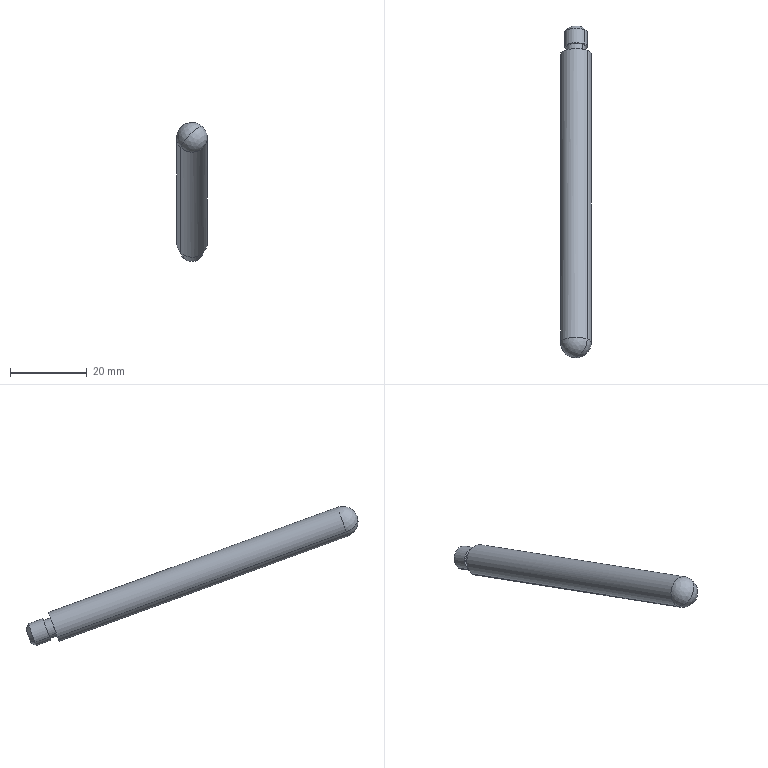Component | SolidWorks | Bipod-1 | 1 solid | 13 faces | box 8 x 86.44 x 36.23 mm | volume 4328 mm3 | cylinder 6 | plane 3 | cone 2 | sphere 2 | commonest cylinder face diameters 8 x2 5 x2 6 x2
build123d program:
from build123d import *

# Parameters (mm, degrees)
FILLET1_R     = 4
CHAMFER1_SIZE = 1


with BuildPart() as part:
    # Sketch1 → Revolve1 (revolve)
    with BuildSketch(Plane.XY, mode=Mode.PRIVATE) as revolve1_sk:
        Polygon((0, 0), (0, 3), (5, 3), (5, 2.5), (7, 2.5), (7, 4), (91, 4), (91, 0), align=None)
    revolve(revolve1_sk.sketch.rotate(Axis((0, 0, 0), (1, 0, 0)), 90), axis=Axis((0, 0, 0), (1, 0, 0)))

    # Fillet1
    fillet1_edges = [part.edges().sort_by_distance(p)[0] for p in [
        (91, 0, -4),
    ]]
    fillet(fillet1_edges, radius=FILLET1_R)

    # Chamfer1
    chamfer1_edges = [part.edges().sort_by_distance(p)[0] for p in [
        (0, 0, -3),
    ]]
    chamfer(chamfer1_edges, length=CHAMFER1_SIZE)


solid = part.part

# Placed as in the assembly
solid = solid.moved(Location((-140.818, 19.624, 1018.001), (160, 0.8472, 90)))
STEP:
#1=CARTESIAN_POINT('',(-5.601,0.7541,40.028));
#2=VERTEX_POINT('',#1);
#3=CARTESIAN_POINT('',(-5.487,0.7911,40.13));
#4=VERTEX_POINT('',#3);
#5=CARTESIAN_POINT('',(-5.544,0.7726,40.079));
#6=DIRECTION('',(-0.,0.9397,-0.342));
#7=DIRECTION('',(0.7279,0.2345,0.6444));
#8=AXIS2_PLACEMENT_3D('',#5,#6,#7);
#9=CIRCLE('',#8,0.07874);
#10=EDGE_CURVE('',#2,#4,#9,.T.);
#11=ORIENTED_EDGE('',*,*,#10,.F.);
#12=CARTESIAN_POINT('',(-5.63,0.7079,40.016));
#13=VERTEX_POINT('',#12);
#14=CARTESIAN_POINT('',(-5.601,0.7541,40.028));
#15=DIRECTION('',(-0.5147,-0.8303,-0.2138));
#16=VECTOR('',#15,39.37);
#17=LINE('',#14,#16);
#18=EDGE_CURVE('',#2,#13,#17,.T.);
#19=ORIENTED_EDGE('',*,*,#18,.T.);
#20=CARTESIAN_POINT('',(-5.458,0.7633,40.168));
#21=VERTEX_POINT('',#20);
#22=CARTESIAN_POINT('',(-5.544,0.7356,40.092));
#23=DIRECTION('',(0.,-0.9397,0.342));
#24=DIRECTION('',(0.7279,0.2345,0.6444));
#25=AXIS2_PLACEMENT_3D('',#22,#23,#24);
#26=CIRCLE('',#25,0.1181);
#27=EDGE_CURVE('',#21,#13,#26,.T.);
#28=ORIENTED_EDGE('',*,*,#27,.F.);
#29=CARTESIAN_POINT('',(-5.487,0.7911,40.13));
#30=DIRECTION('',(0.5147,-0.4986,0.6975));
#31=VECTOR('',#30,39.37);
#32=LINE('',#29,#31);
#33=EDGE_CURVE('',#4,#21,#32,.T.);
#34=ORIENTED_EDGE('',*,*,#33,.F.);
#35=EDGE_LOOP('',(#11,#19,#28,#34));
#36=FACE_OUTER_BOUND('',#35,.T.);
#37=CARTESIAN_POINT('',(-5.544,0.7726,40.079));
#38=DIRECTION('',(0.,-0.9397,0.342));
#39=DIRECTION('',(0.7279,0.2345,0.6444));
#40=AXIS2_PLACEMENT_3D('',#37,#38,#39);
#41=CONICAL_SURFACE('',#40,0.07874,0.7854);
#42=ADVANCED_FACE('',(#36),#41,.T.);
#43=CARTESIAN_POINT('',(-5.544,-2.594,41.304));
#44=VERTEX_POINT('',#43);
#45=CARTESIAN_POINT('',(-5.659,-2.483,41.149));
#46=VERTEX_POINT('',#45);
#47=CARTESIAN_POINT('',(-5.544,-2.446,41.25));
#48=DIRECTION('',(0.6857,-0.2489,-0.684));
#49=DIRECTION('',(-0.7062,0.,-0.708));
#50=AXIS2_PLACEMENT_3D('',#47,#48,#49);
#51=CIRCLE('',#50,0.1575);
#52=EDGE_CURVE('',#44,#46,#51,.T.);
#53=ORIENTED_EDGE('',*,*,#52,.F.);
#54=CARTESIAN_POINT('',(-5.429,-2.409,41.352));
#55=VERTEX_POINT('',#54);
#56=CARTESIAN_POINT('',(-5.544,-2.446,41.25));
#57=DIRECTION('',(-0.6857,0.2489,0.684));
#58=DIRECTION('',(0.7062,0.,0.708));
#59=AXIS2_PLACEMENT_3D('',#56,#57,#58);
#60=CIRCLE('',#59,0.1575);
#61=EDGE_CURVE('',#44,#55,#60,.T.);
#62=ORIENTED_EDGE('',*,*,#61,.T.);
#63=CARTESIAN_POINT('',(-5.544,-2.446,41.25));
#64=DIRECTION('',(-0.,0.9397,-0.342));
#65=DIRECTION('',(-0.7279,-0.2345,-0.6444));
#66=AXIS2_PLACEMENT_3D('',#63,#64,#65);
#67=CIRCLE('',#66,0.1575);
#68=EDGE_CURVE('',#46,#55,#67,.T.);
#69=ORIENTED_EDGE('',*,*,#68,.F.);
#70=EDGE_LOOP('',(#53,#62,#69));
#71=FACE_OUTER_BOUND('',#70,.T.);
#72=CARTESIAN_POINT('',(-5.544,-2.446,41.25));
#73=DIRECTION('',(-0.6857,0.2489,0.684));
#74=DIRECTION('',(-0.7279,-0.2345,-0.6444));
#75=AXIS2_PLACEMENT_3D('',#72,#73,#74);
#76=SPHERICAL_SURFACE('',#75,0.1575);
#77=ADVANCED_FACE('',(#71),#76,.T.);
#78=ORIENTED_EDGE('',*,*,#68,.T.);
#79=CARTESIAN_POINT('',(-5.429,0.5506,40.275));
#80=VERTEX_POINT('',#79);
#81=CARTESIAN_POINT('',(-5.429,0.8095,40.18));
#82=DIRECTION('',(-0.,0.9397,-0.342));
#83=VECTOR('',#82,39.37);
#84=LINE('',#81,#83);
#85=EDGE_CURVE('',#55,#80,#84,.T.);
#86=ORIENTED_EDGE('',*,*,#85,.T.);
#87=CARTESIAN_POINT('',(-5.659,0.4767,40.072));
#88=VERTEX_POINT('',#87);
#89=CARTESIAN_POINT('',(-5.544,0.5136,40.173));
#90=DIRECTION('',(-0.,0.9397,-0.342));
#91=DIRECTION('',(-0.7279,-0.2345,-0.6444));
#92=AXIS2_PLACEMENT_3D('',#89,#90,#91);
#93=CIRCLE('',#92,0.1575);
#94=EDGE_CURVE('',#88,#80,#93,.T.);
#95=ORIENTED_EDGE('',*,*,#94,.F.);
#96=CARTESIAN_POINT('',(-5.659,0.7357,39.977));
#97=DIRECTION('',(-0.,0.9397,-0.342));
#98=VECTOR('',#97,39.37);
#99=LINE('',#96,#98);
#100=EDGE_CURVE('',#46,#88,#99,.T.);
#101=ORIENTED_EDGE('',*,*,#100,.F.);
#102=EDGE_LOOP('',(#78,#86,#95,#101));
#103=FACE_OUTER_BOUND('',#102,.T.);
#104=CARTESIAN_POINT('',(-5.544,0.7726,40.079));
#105=DIRECTION('',(-0.,0.9397,-0.342));
#106=DIRECTION('',(-0.7279,-0.2345,-0.6444));
#107=AXIS2_PLACEMENT_3D('',#104,#105,#106);
#108=CYLINDRICAL_SURFACE('',#107,0.1575);
#109=ADVANCED_FACE('',(#103),#108,.T.);
#110=CARTESIAN_POINT('',(-5.616,0.4905,40.11));
#111=VERTEX_POINT('',#110);
#112=CARTESIAN_POINT('',(-5.472,0.5367,40.236));
#113=VERTEX_POINT('',#112);
#114=CARTESIAN_POINT('',(-5.544,0.5136,40.173));
#115=DIRECTION('',(-0.,0.9397,-0.342));
#116=DIRECTION('',(-0.7279,-0.2345,-0.6444));
#117=AXIS2_PLACEMENT_3D('',#114,#115,#116);
#118=CIRCLE('',#117,0.09843);
#119=EDGE_CURVE('',#111,#113,#118,.T.);
#120=ORIENTED_EDGE('',*,*,#119,.T.);
#121=CARTESIAN_POINT('',(-5.472,0.6107,40.21));
#122=VERTEX_POINT('',#121);
#123=CARTESIAN_POINT('',(-5.472,0.7957,40.142));
#124=DIRECTION('',(-0.,0.9397,-0.342));
#125=VECTOR('',#124,39.37);
#126=LINE('',#123,#125);
#127=EDGE_CURVE('',#113,#122,#126,.T.);
#128=ORIENTED_EDGE('',*,*,#127,.T.);
#129=CARTESIAN_POINT('',(-5.616,0.5645,40.083));
#130=VERTEX_POINT('',#129);
#131=CARTESIAN_POINT('',(-5.544,0.5876,40.146));
#132=DIRECTION('',(-0.,0.9397,-0.342));
#133=DIRECTION('',(-0.7279,-0.2345,-0.6444));
#134=AXIS2_PLACEMENT_3D('',#131,#132,#133);
#135=CIRCLE('',#134,0.09843);
#136=EDGE_CURVE('',#130,#122,#135,.T.);
#137=ORIENTED_EDGE('',*,*,#136,.F.);
#138=CARTESIAN_POINT('',(-5.616,0.7495,40.015));
#139=DIRECTION('',(-0.,0.9397,-0.342));
#140=VECTOR('',#139,39.37);
#141=LINE('',#138,#140);
#142=EDGE_CURVE('',#111,#130,#141,.T.);
#143=ORIENTED_EDGE('',*,*,#142,.F.);
#144=EDGE_LOOP('',(#120,#128,#137,#143));
#145=FACE_OUTER_BOUND('',#144,.T.);
#146=CARTESIAN_POINT('',(-5.544,0.7726,40.079));
#147=DIRECTION('',(-0.,0.9397,-0.342));
#148=DIRECTION('',(-0.7279,-0.2345,-0.6444));
#149=AXIS2_PLACEMENT_3D('',#146,#147,#148);
#150=CYLINDRICAL_SURFACE('',#149,0.09843);
#151=ADVANCED_FACE('',(#145),#150,.T.);
#152=CARTESIAN_POINT('',(-5.63,0.5599,40.07));
#153=VERTEX_POINT('',#152);
#154=CARTESIAN_POINT('',(-5.458,0.6153,40.222));
#155=VERTEX_POINT('',#154);
#156=CARTESIAN_POINT('',(-5.544,0.5876,40.146));
#157=DIRECTION('',(-0.,0.9397,-0.342));
#158=DIRECTION('',(-0.7279,-0.2345,-0.6444));
#159=AXIS2_PLACEMENT_3D('',#156,#157,#158);
#160=CIRCLE('',#159,0.1181);
#161=EDGE_CURVE('',#153,#155,#160,.T.);
#162=ORIENTED_EDGE('',*,*,#161,.T.);
#163=CARTESIAN_POINT('',(-5.458,0.8003,40.155));
#164=DIRECTION('',(-0.,0.9397,-0.342));
#165=VECTOR('',#164,39.37);
#166=LINE('',#163,#165);
#167=EDGE_CURVE('',#155,#21,#166,.T.);
#168=ORIENTED_EDGE('',*,*,#167,.T.);
#169=ORIENTED_EDGE('',*,*,#27,.T.);
#170=CARTESIAN_POINT('',(-5.63,0.7449,40.003));
#171=DIRECTION('',(-0.,0.9397,-0.342));
#172=VECTOR('',#171,39.37);
#173=LINE('',#170,#172);
#174=EDGE_CURVE('',#153,#13,#173,.T.);
#175=ORIENTED_EDGE('',*,*,#174,.F.);
#176=EDGE_LOOP('',(#162,#168,#169,#175));
#177=FACE_OUTER_BOUND('',#176,.T.);
#178=CARTESIAN_POINT('',(-5.544,0.7726,40.079));
#179=DIRECTION('',(-0.,0.9397,-0.342));
#180=DIRECTION('',(-0.7279,-0.2345,-0.6444));
#181=AXIS2_PLACEMENT_3D('',#178,#179,#180);
#182=CYLINDRICAL_SURFACE('',#181,0.1181);
#183=ADVANCED_FACE('',(#177),#182,.T.);
#184=CARTESIAN_POINT('',(-5.544,0.7726,40.079));
#185=DIRECTION('',(-0.,0.9397,-0.342));
#186=DIRECTION('',(0.7279,0.2345,0.6444));
#187=AXIS2_PLACEMENT_3D('',#184,#185,#186);
#188=CIRCLE('',#187,0.07874);
#189=EDGE_CURVE('',#4,#2,#188,.T.);
#190=ORIENTED_EDGE('',*,*,#189,.T.);
#191=ORIENTED_EDGE('',*,*,#10,.T.);
#192=EDGE_LOOP('',(#190,#191));
#193=FACE_OUTER_BOUND('',#192,.T.);
#194=CARTESIAN_POINT('',(-5.544,0.7726,40.079));
#195=DIRECTION('',(-0.,-0.9397,0.342));
#196=DIRECTION('',(0.7279,0.2345,0.6444));
#197=AXIS2_PLACEMENT_3D('',#194,#195,#196);
#198=PLANE('',#197);
#199=ADVANCED_FACE('',(#193),#198,.F.);
#200=ORIENTED_EDGE('',*,*,#167,.F.);
#201=CARTESIAN_POINT('',(-5.544,0.5876,40.146));
#202=DIRECTION('',(-0.,0.9397,-0.342));
#203=DIRECTION('',(-0.7279,-0.2345,-0.6444));
#204=AXIS2_PLACEMENT_3D('',#201,#202,#203);
#205=CIRCLE('',#204,0.1181);
#206=EDGE_CURVE('',#155,#153,#205,.T.);
#207=ORIENTED_EDGE('',*,*,#206,.T.);
#208=ORIENTED_EDGE('',*,*,#174,.T.);
#209=CARTESIAN_POINT('',(-5.544,0.7356,40.092));
#210=DIRECTION('',(0.,-0.9397,0.342));
#211=DIRECTION('',(0.7279,0.2345,0.6444));
#212=AXIS2_PLACEMENT_3D('',#209,#210,#211);
#213=CIRCLE('',#212,0.1181);
#214=EDGE_CURVE('',#13,#21,#213,.T.);
#215=ORIENTED_EDGE('',*,*,#214,.T.);
#216=EDGE_LOOP('',(#200,#207,#208,#215));
#217=FACE_OUTER_BOUND('',#216,.T.);
#218=CARTESIAN_POINT('',(-5.544,0.7726,40.079));
#219=DIRECTION('',(-0.,0.9397,-0.342));
#220=DIRECTION('',(-0.7279,-0.2345,-0.6444));
#221=AXIS2_PLACEMENT_3D('',#218,#219,#220);
#222=CYLINDRICAL_SURFACE('',#221,0.1181);
#223=ADVANCED_FACE('',(#217),#222,.T.);
#224=ORIENTED_EDGE('',*,*,#161,.F.);
#225=ORIENTED_EDGE('',*,*,#206,.F.);
#226=EDGE_LOOP('',(#224,#225));
#227=FACE_OUTER_BOUND('',#226,.T.);
#228=ORIENTED_EDGE('',*,*,#136,.T.);
#229=CARTESIAN_POINT('',(-5.544,0.5876,40.146));
#230=DIRECTION('',(-0.,0.9397,-0.342));
#231=DIRECTION('',(-0.7279,-0.2345,-0.6444));
#232=AXIS2_PLACEMENT_3D('',#229,#230,#231);
#233=CIRCLE('',#232,0.09843);
#234=EDGE_CURVE('',#122,#130,#233,.T.);
#235=ORIENTED_EDGE('',*,*,#234,.T.);
#236=EDGE_LOOP('',(#228,#235));
#237=FACE_BOUND('',#236,.T.);
#238=CARTESIAN_POINT('',(-5.625,0.617,40.227));
#239=DIRECTION('',(0.,0.9397,-0.342));
#240=DIRECTION('',(-0.7279,-0.2345,-0.6444));
#241=AXIS2_PLACEMENT_3D('',#238,#239,#240);
#242=PLANE('',#241);
#243=ADVANCED_FACE('',(#227,#237),#242,.F.);
#244=ORIENTED_EDGE('',*,*,#127,.F.);
#245=CARTESIAN_POINT('',(-5.544,0.5136,40.173));
#246=DIRECTION('',(-0.,0.9397,-0.342));
#247=DIRECTION('',(-0.7279,-0.2345,-0.6444));
#248=AXIS2_PLACEMENT_3D('',#245,#246,#247);
#249=CIRCLE('',#248,0.09843);
#250=EDGE_CURVE('',#113,#111,#249,.T.);
#251=ORIENTED_EDGE('',*,*,#250,.T.);
#252=ORIENTED_EDGE('',*,*,#142,.T.);
#253=ORIENTED_EDGE('',*,*,#234,.F.);
#254=EDGE_LOOP('',(#244,#251,#252,#253));
#255=FACE_OUTER_BOUND('',#254,.T.);
#256=CARTESIAN_POINT('',(-5.544,0.7726,40.079));
#257=DIRECTION('',(-0.,0.9397,-0.342));
#258=DIRECTION('',(-0.7279,-0.2345,-0.6444));
#259=AXIS2_PLACEMENT_3D('',#256,#257,#258);
#260=CYLINDRICAL_SURFACE('',#259,0.09843);
#261=ADVANCED_FACE('',(#255),#260,.T.);
#262=ORIENTED_EDGE('',*,*,#119,.F.);
#263=ORIENTED_EDGE('',*,*,#250,.F.);
#264=EDGE_LOOP('',(#262,#263));
#265=FACE_BOUND('',#264,.T.);
#266=ORIENTED_EDGE('',*,*,#94,.T.);
#267=CARTESIAN_POINT('',(-5.544,0.5136,40.173));
#268=DIRECTION('',(-0.,0.9397,-0.342));
#269=DIRECTION('',(-0.7279,-0.2345,-0.6444));
#270=AXIS2_PLACEMENT_3D('',#267,#268,#269);
#271=CIRCLE('',#270,0.1575);
#272=EDGE_CURVE('',#80,#88,#271,.T.);
#273=ORIENTED_EDGE('',*,*,#272,.T.);
#274=EDGE_LOOP('',(#266,#273));
#275=FACE_OUTER_BOUND('',#274,.T.);
#276=CARTESIAN_POINT('',(-5.611,0.5381,40.24));
#277=DIRECTION('',(-0.,-0.9397,0.342));
#278=DIRECTION('',(0.7279,0.2345,0.6444));
#279=AXIS2_PLACEMENT_3D('',#276,#277,#278);
#280=PLANE('',#279);
#281=ADVANCED_FACE('',(#265,#275),#280,.F.);
#282=ORIENTED_EDGE('',*,*,#85,.F.);
#283=CARTESIAN_POINT('',(-5.544,-2.446,41.25));
#284=DIRECTION('',(-0.,0.9397,-0.342));
#285=DIRECTION('',(-0.7279,-0.2345,-0.6444));
#286=AXIS2_PLACEMENT_3D('',#283,#284,#285);
#287=CIRCLE('',#286,0.1575);
#288=EDGE_CURVE('',#55,#46,#287,.T.);
#289=ORIENTED_EDGE('',*,*,#288,.T.);
#290=ORIENTED_EDGE('',*,*,#100,.T.);
#291=ORIENTED_EDGE('',*,*,#272,.F.);
#292=EDGE_LOOP('',(#282,#289,#290,#291));
#293=FACE_OUTER_BOUND('',#292,.T.);
#294=CARTESIAN_POINT('',(-5.544,0.7726,40.079));
#295=DIRECTION('',(-0.,0.9397,-0.342));
#296=DIRECTION('',(-0.7279,-0.2345,-0.6444));
#297=AXIS2_PLACEMENT_3D('',#294,#295,#296);
#298=CYLINDRICAL_SURFACE('',#297,0.1575);
#299=ADVANCED_FACE('',(#293),#298,.T.);
#300=ORIENTED_EDGE('',*,*,#61,.F.);
#301=ORIENTED_EDGE('',*,*,#52,.T.);
#302=ORIENTED_EDGE('',*,*,#288,.F.);
#303=EDGE_LOOP('',(#300,#301,#302));
#304=FACE_OUTER_BOUND('',#303,.T.);
#305=CARTESIAN_POINT('',(-5.544,-2.446,41.25));
#306=DIRECTION('',(-0.6857,0.2489,0.684));
#307=DIRECTION('',(-0.7279,-0.2345,-0.6444));
#308=AXIS2_PLACEMENT_3D('',#305,#306,#307);
#309=SPHERICAL_SURFACE('',#308,0.1575);
#310=ADVANCED_FACE('',(#304),#309,.T.);
#311=ORIENTED_EDGE('',*,*,#18,.F.);
#312=ORIENTED_EDGE('',*,*,#189,.F.);
#313=ORIENTED_EDGE('',*,*,#33,.T.);
#314=ORIENTED_EDGE('',*,*,#214,.F.);
#315=EDGE_LOOP('',(#311,#312,#313,#314));
#316=FACE_OUTER_BOUND('',#315,.T.);
#317=CARTESIAN_POINT('',(-5.544,0.7726,40.079));
#318=DIRECTION('',(0.,-0.9397,0.342));
#319=DIRECTION('',(0.7279,0.2345,0.6444));
#320=AXIS2_PLACEMENT_3D('',#317,#318,#319);
#321=CONICAL_SURFACE('',#320,0.07874,0.7854);
#322=ADVANCED_FACE('',(#316),#321,.T.);
#323=CLOSED_SHELL('',(#42,#77,#109,#151,#183,#199,#223,#243,#261,#281,#299,#310,#322));
#324=MANIFOLD_SOLID_BREP('',#323);
#325=CARTESIAN_POINT('',(0.,0.,0.));
#326=DIRECTION('',(0.,0.,1.));
#327=DIRECTION('',(1.,0.,0.));
#328=AXIS2_PLACEMENT_3D('',#325,#326,#327);
#329=(LENGTH_UNIT()NAMED_UNIT(*)SI_UNIT($,.METRE.));
#330=LENGTH_MEASURE_WITH_UNIT(LENGTH_MEASURE(0.0254),#329);
#331=DIMENSIONAL_EXPONENTS(1.,0.,0.,0.,0.,0.,0.);
#332=(CONVERSION_BASED_UNIT('',#330)LENGTH_UNIT()NAMED_UNIT(#331));
#333=UNCERTAINTY_MEASURE_WITH_UNIT(LENGTH_MEASURE(0.00001),#332,'','');
#334=(NAMED_UNIT(*)PLANE_ANGLE_UNIT()SI_UNIT($,.RADIAN.));
#335=(NAMED_UNIT(*)SI_UNIT($,.STERADIAN.)SOLID_ANGLE_UNIT());
#336=(GEOMETRIC_REPRESENTATION_CONTEXT(3)GLOBAL_UNCERTAINTY_ASSIGNED_CONTEXT((#333))GLOBAL_UNIT_ASSIGNED_CONTEXT((#332,#334,#335))REPRESENTATION_CONTEXT('',''));
#337=ADVANCED_BREP_SHAPE_REPRESENTATION('',(#324,#328),#336);
#338=COLOUR_RGB('',0.7922,0.8196,0.9333);
#339=FILL_AREA_STYLE_COLOUR('',#338);
#340=FILL_AREA_STYLE('',(#339));
#341=SURFACE_STYLE_FILL_AREA(#340);
#342=SURFACE_SIDE_STYLE('',(#341));
#343=SURFACE_STYLE_USAGE(.BOTH.,#342);
#344=PRESENTATION_STYLE_ASSIGNMENT((#343));
#345=STYLED_ITEM('',(#344),#324);
#346=(LENGTH_UNIT()NAMED_UNIT(*)SI_UNIT($,.METRE.));
#347=LENGTH_MEASURE_WITH_UNIT(LENGTH_MEASURE(0.0254),#346);
#348=DIMENSIONAL_EXPONENTS(1.,0.,0.,0.,0.,0.,0.);
#349=(CONVERSION_BASED_UNIT('',#347)LENGTH_UNIT()NAMED_UNIT(#348));
#350=UNCERTAINTY_MEASURE_WITH_UNIT(LENGTH_MEASURE(0.00001),#349,'','');
#351=(NAMED_UNIT(*)PLANE_ANGLE_UNIT()SI_UNIT($,.RADIAN.));
#352=(NAMED_UNIT(*)SI_UNIT($,.STERADIAN.)SOLID_ANGLE_UNIT());
#353=(GEOMETRIC_REPRESENTATION_CONTEXT(3)GLOBAL_UNCERTAINTY_ASSIGNED_CONTEXT((#350))GLOBAL_UNIT_ASSIGNED_CONTEXT((#349,#351,#352))REPRESENTATION_CONTEXT('',''));
#354=MECHANICAL_DESIGN_GEOMETRIC_PRESENTATION_REPRESENTATION('',(#345),#353);
#355=PRESENTATION_LAYER_ASSIGNMENT('','',(#345));